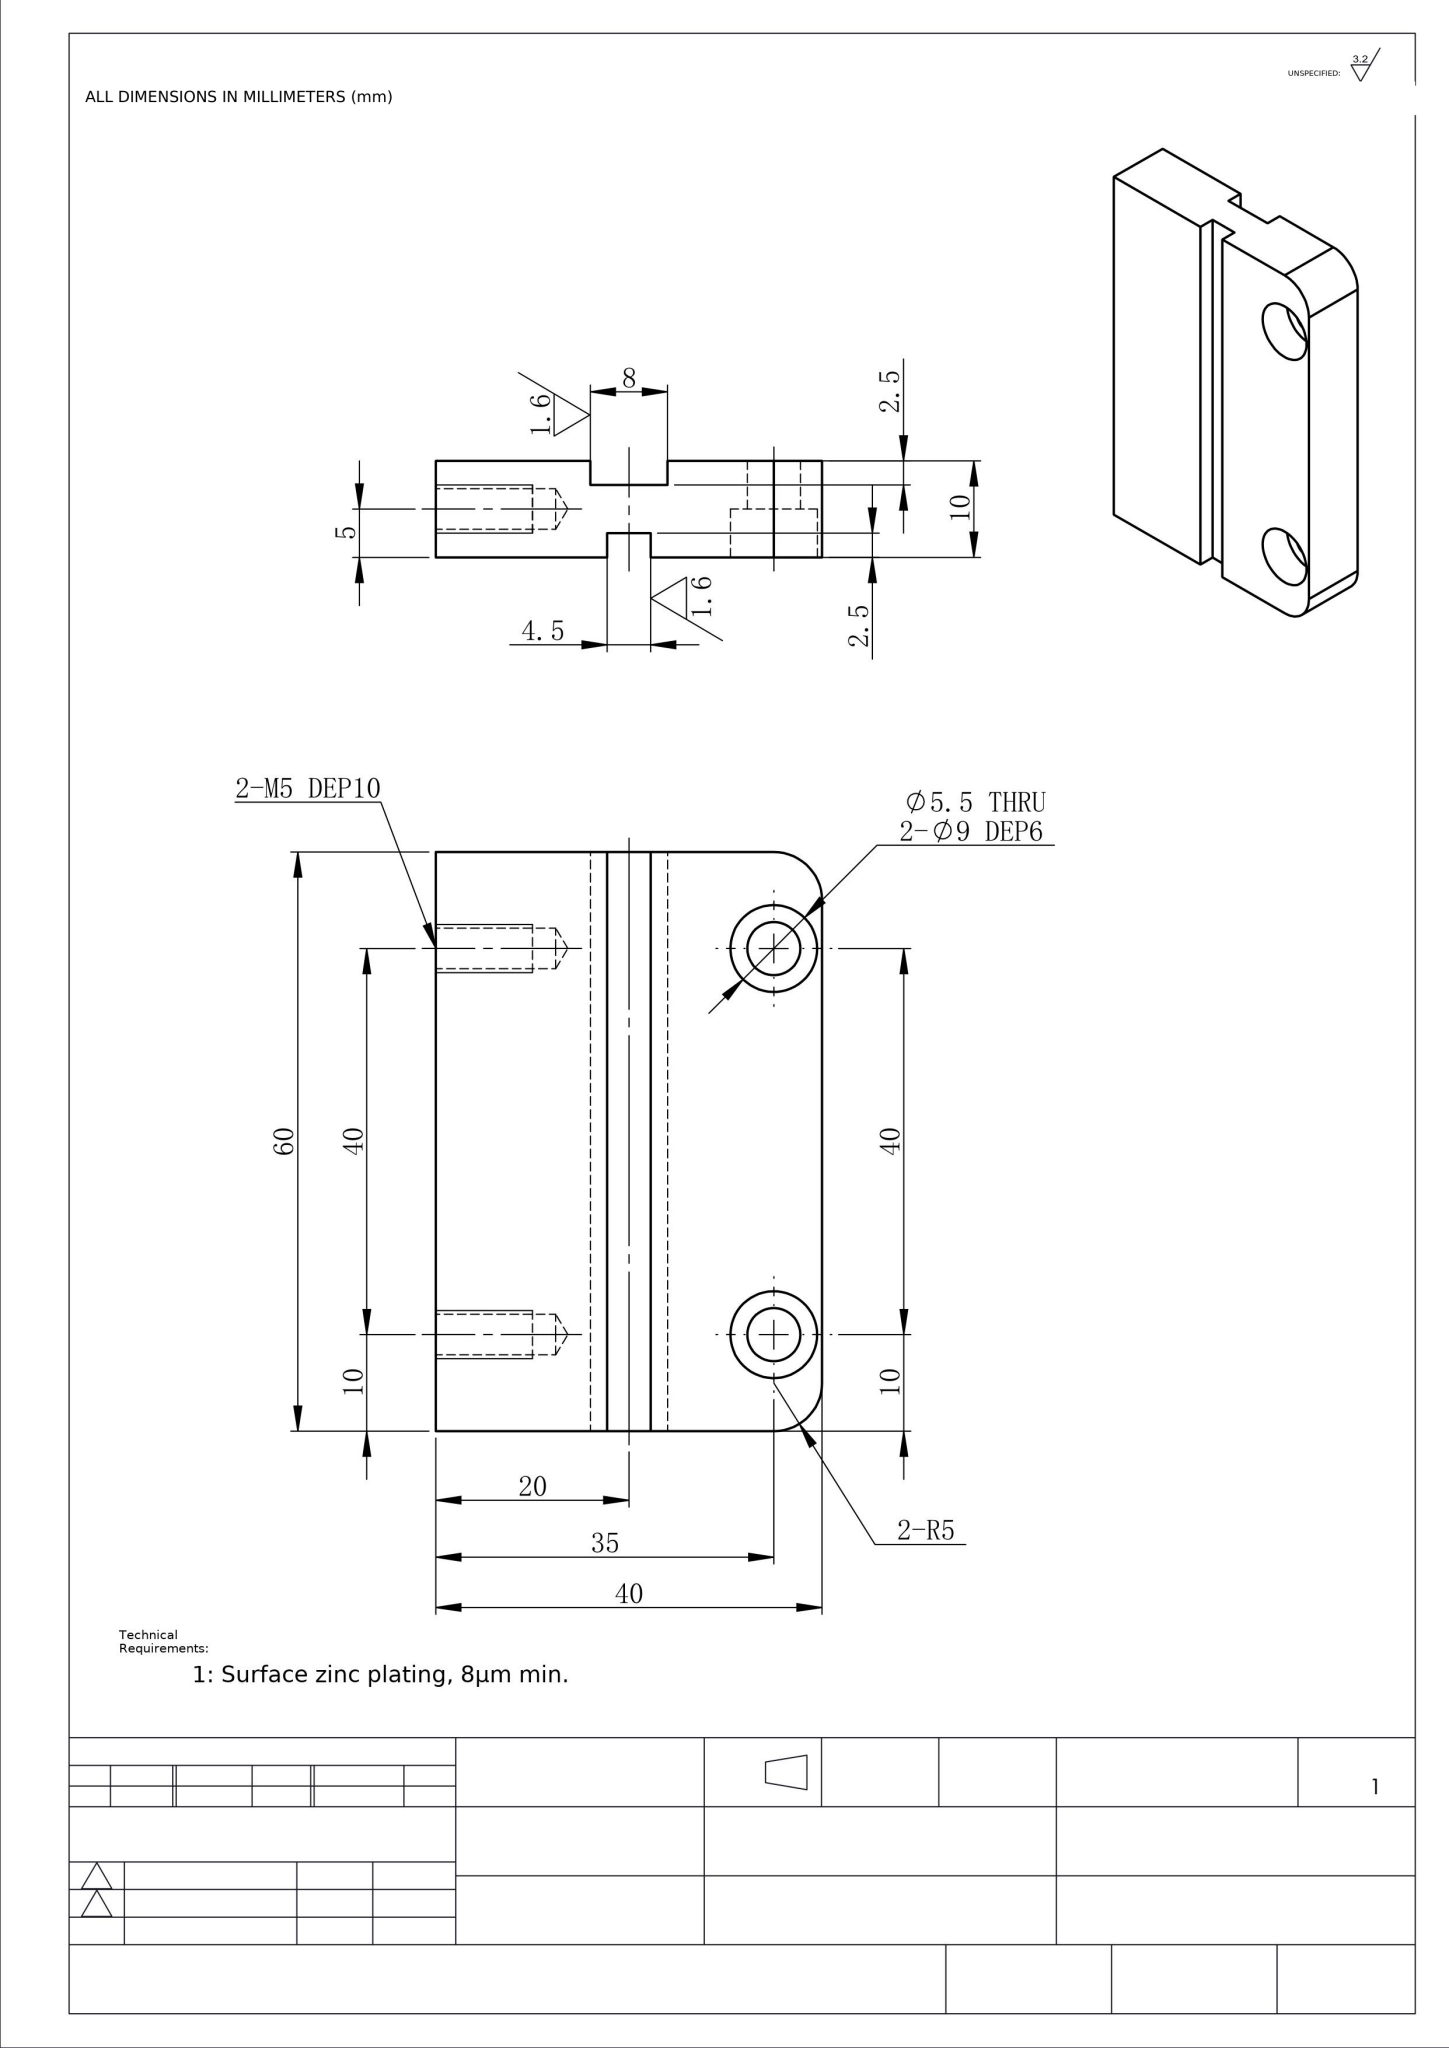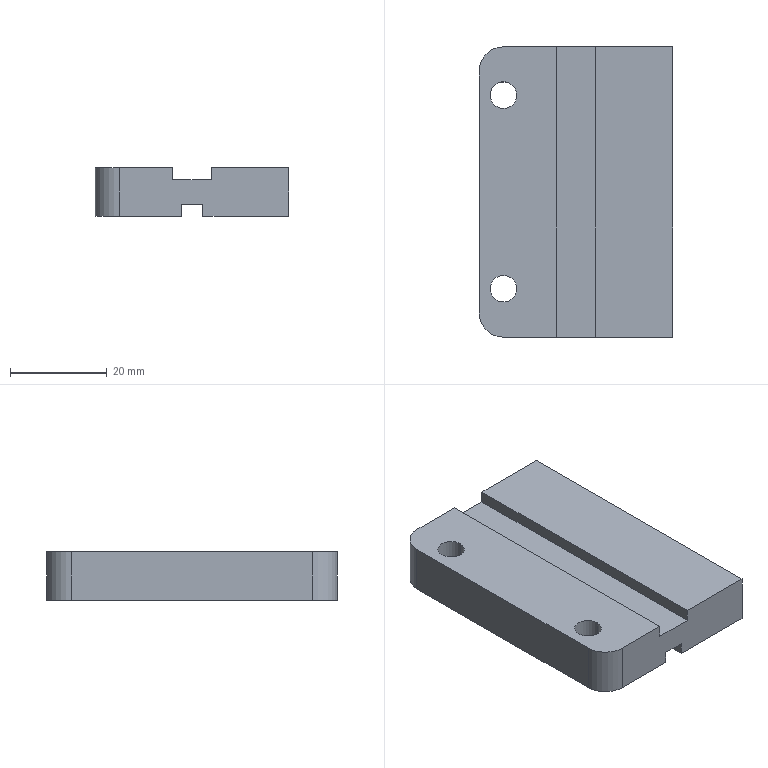Part | NX | mm | 1 solid | 34 faces | box 40 x 60 x 10 mm | volume 20789 mm3 | plane 16 | cylinder 14 | cone 4 | commonest cylinder face diameters 4.2 x4 5.5 x4 9 x4 10 x2